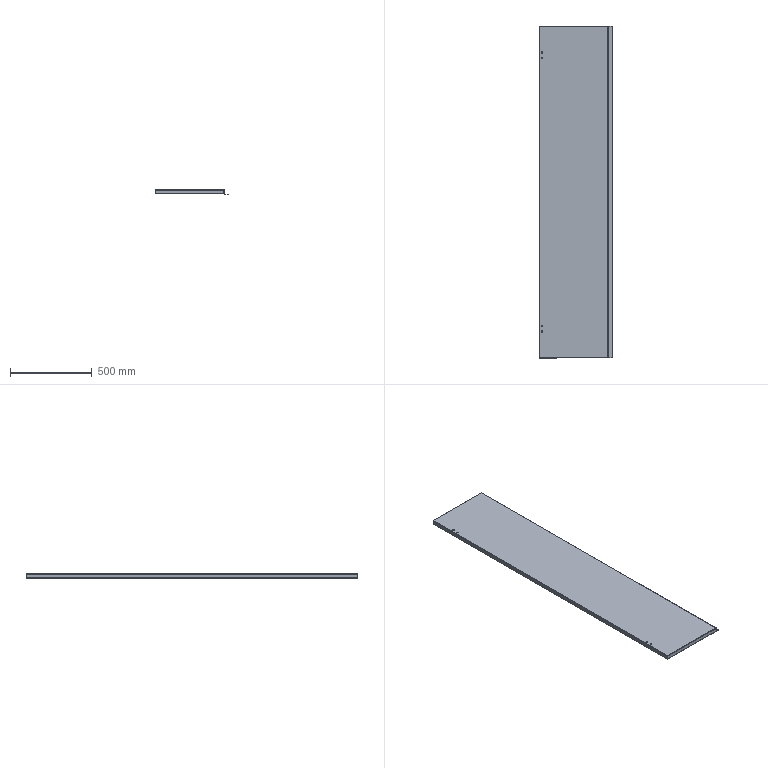Component | SolidWorks | 36ResistorLeftFrontDoor-1 | 1 solid | 72 faces | volume 2090647 mm3 | plane 40 | cylinder 24 | spline 8 | commonest cylinder face diameters 10 x8 2 x8 6 x8